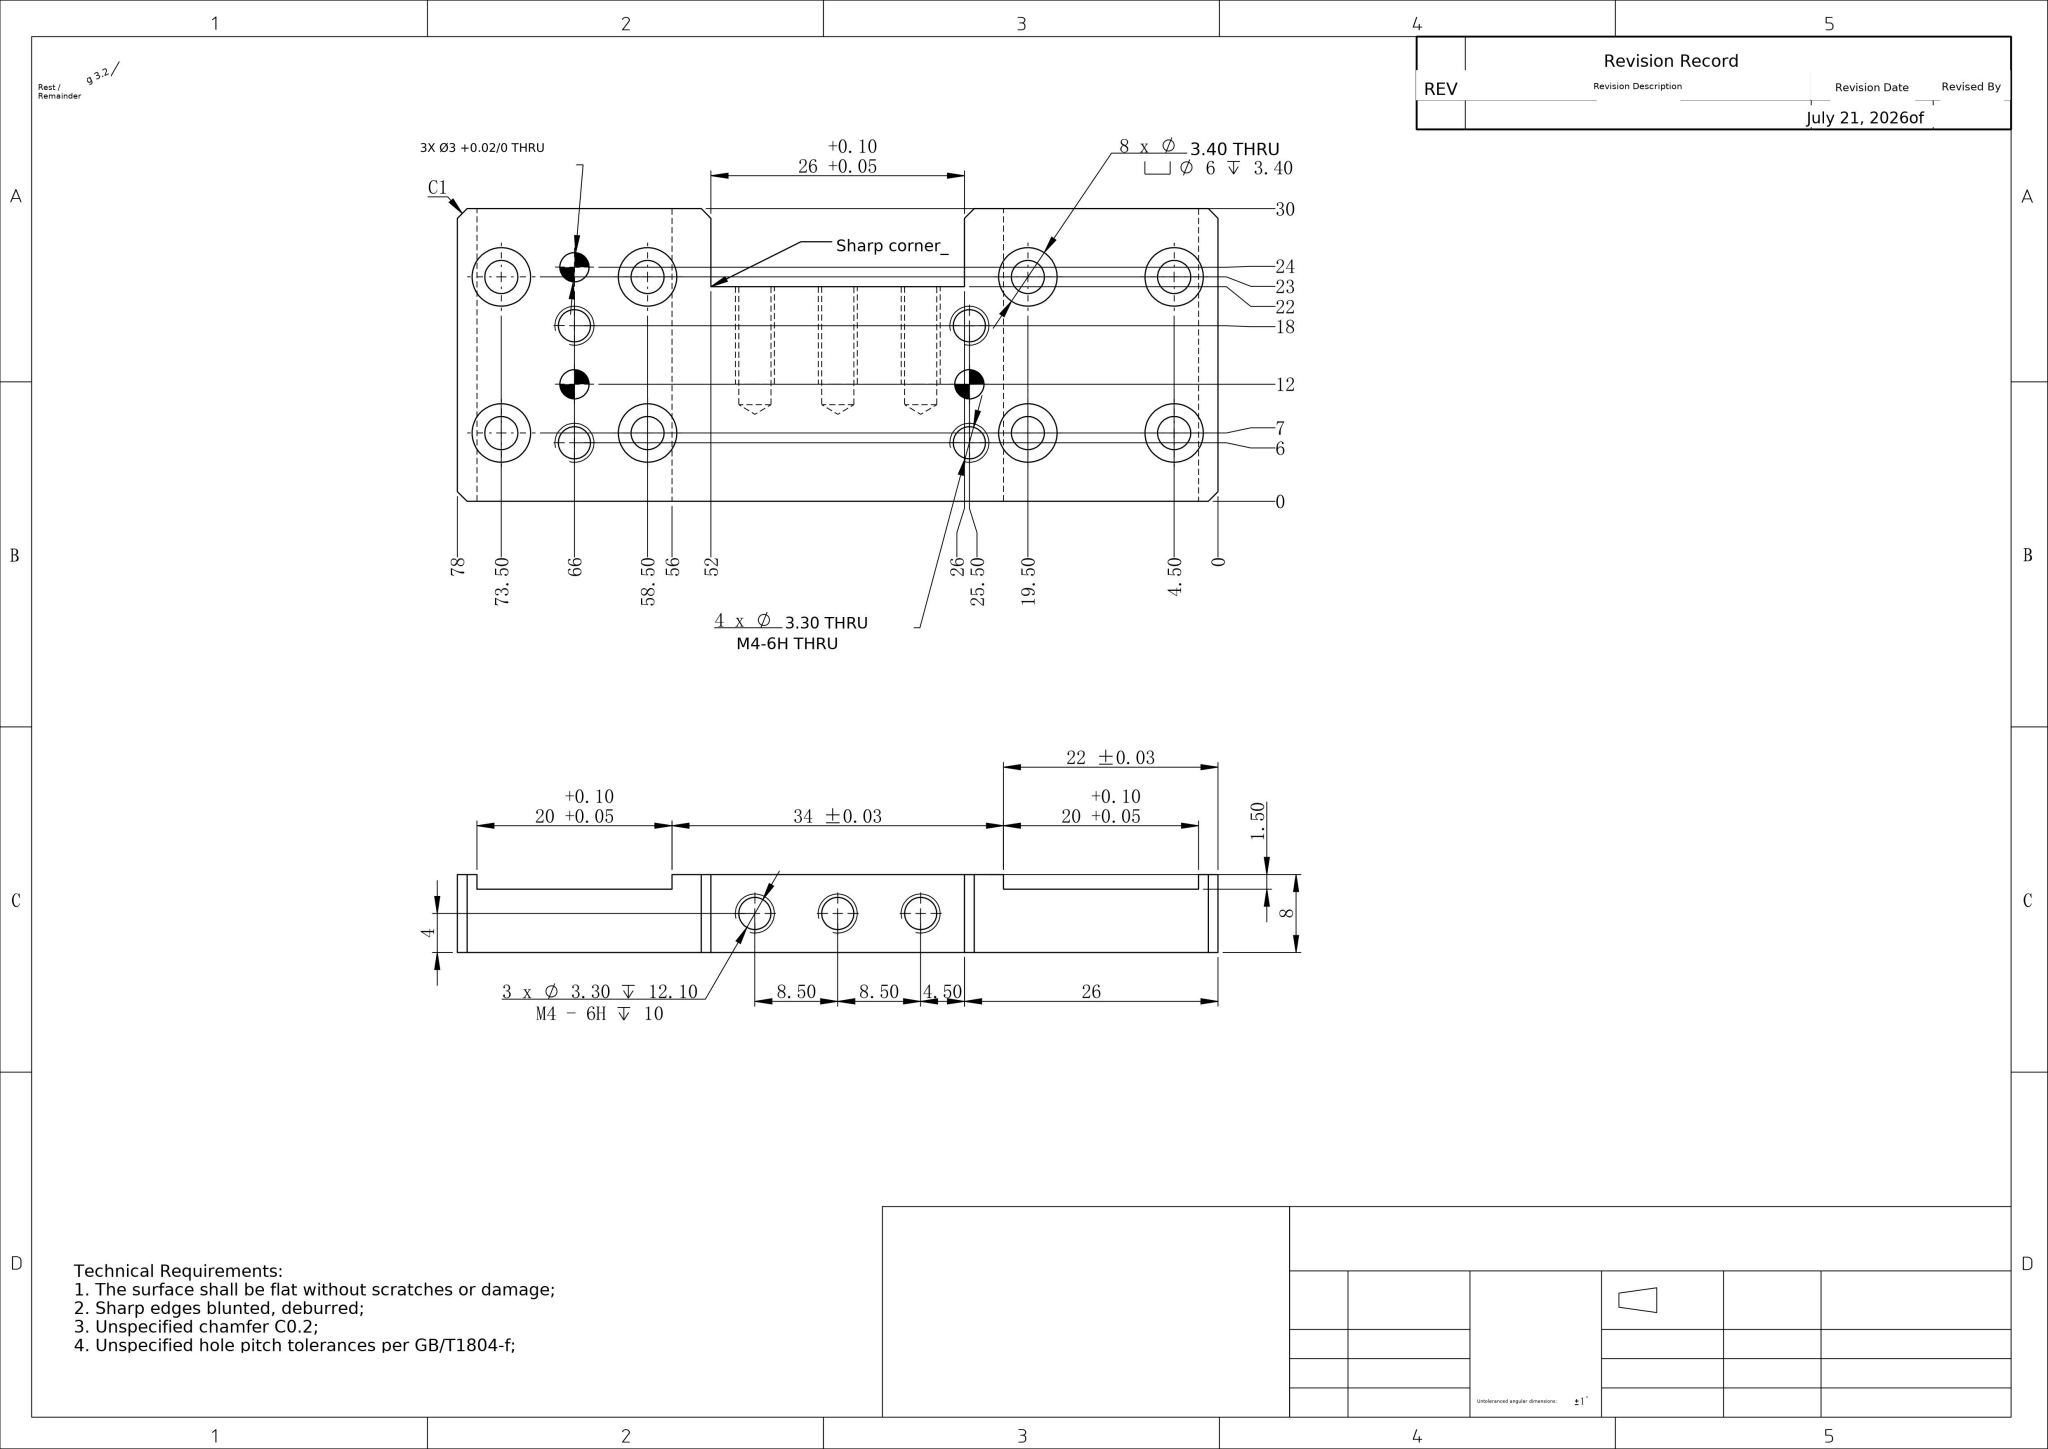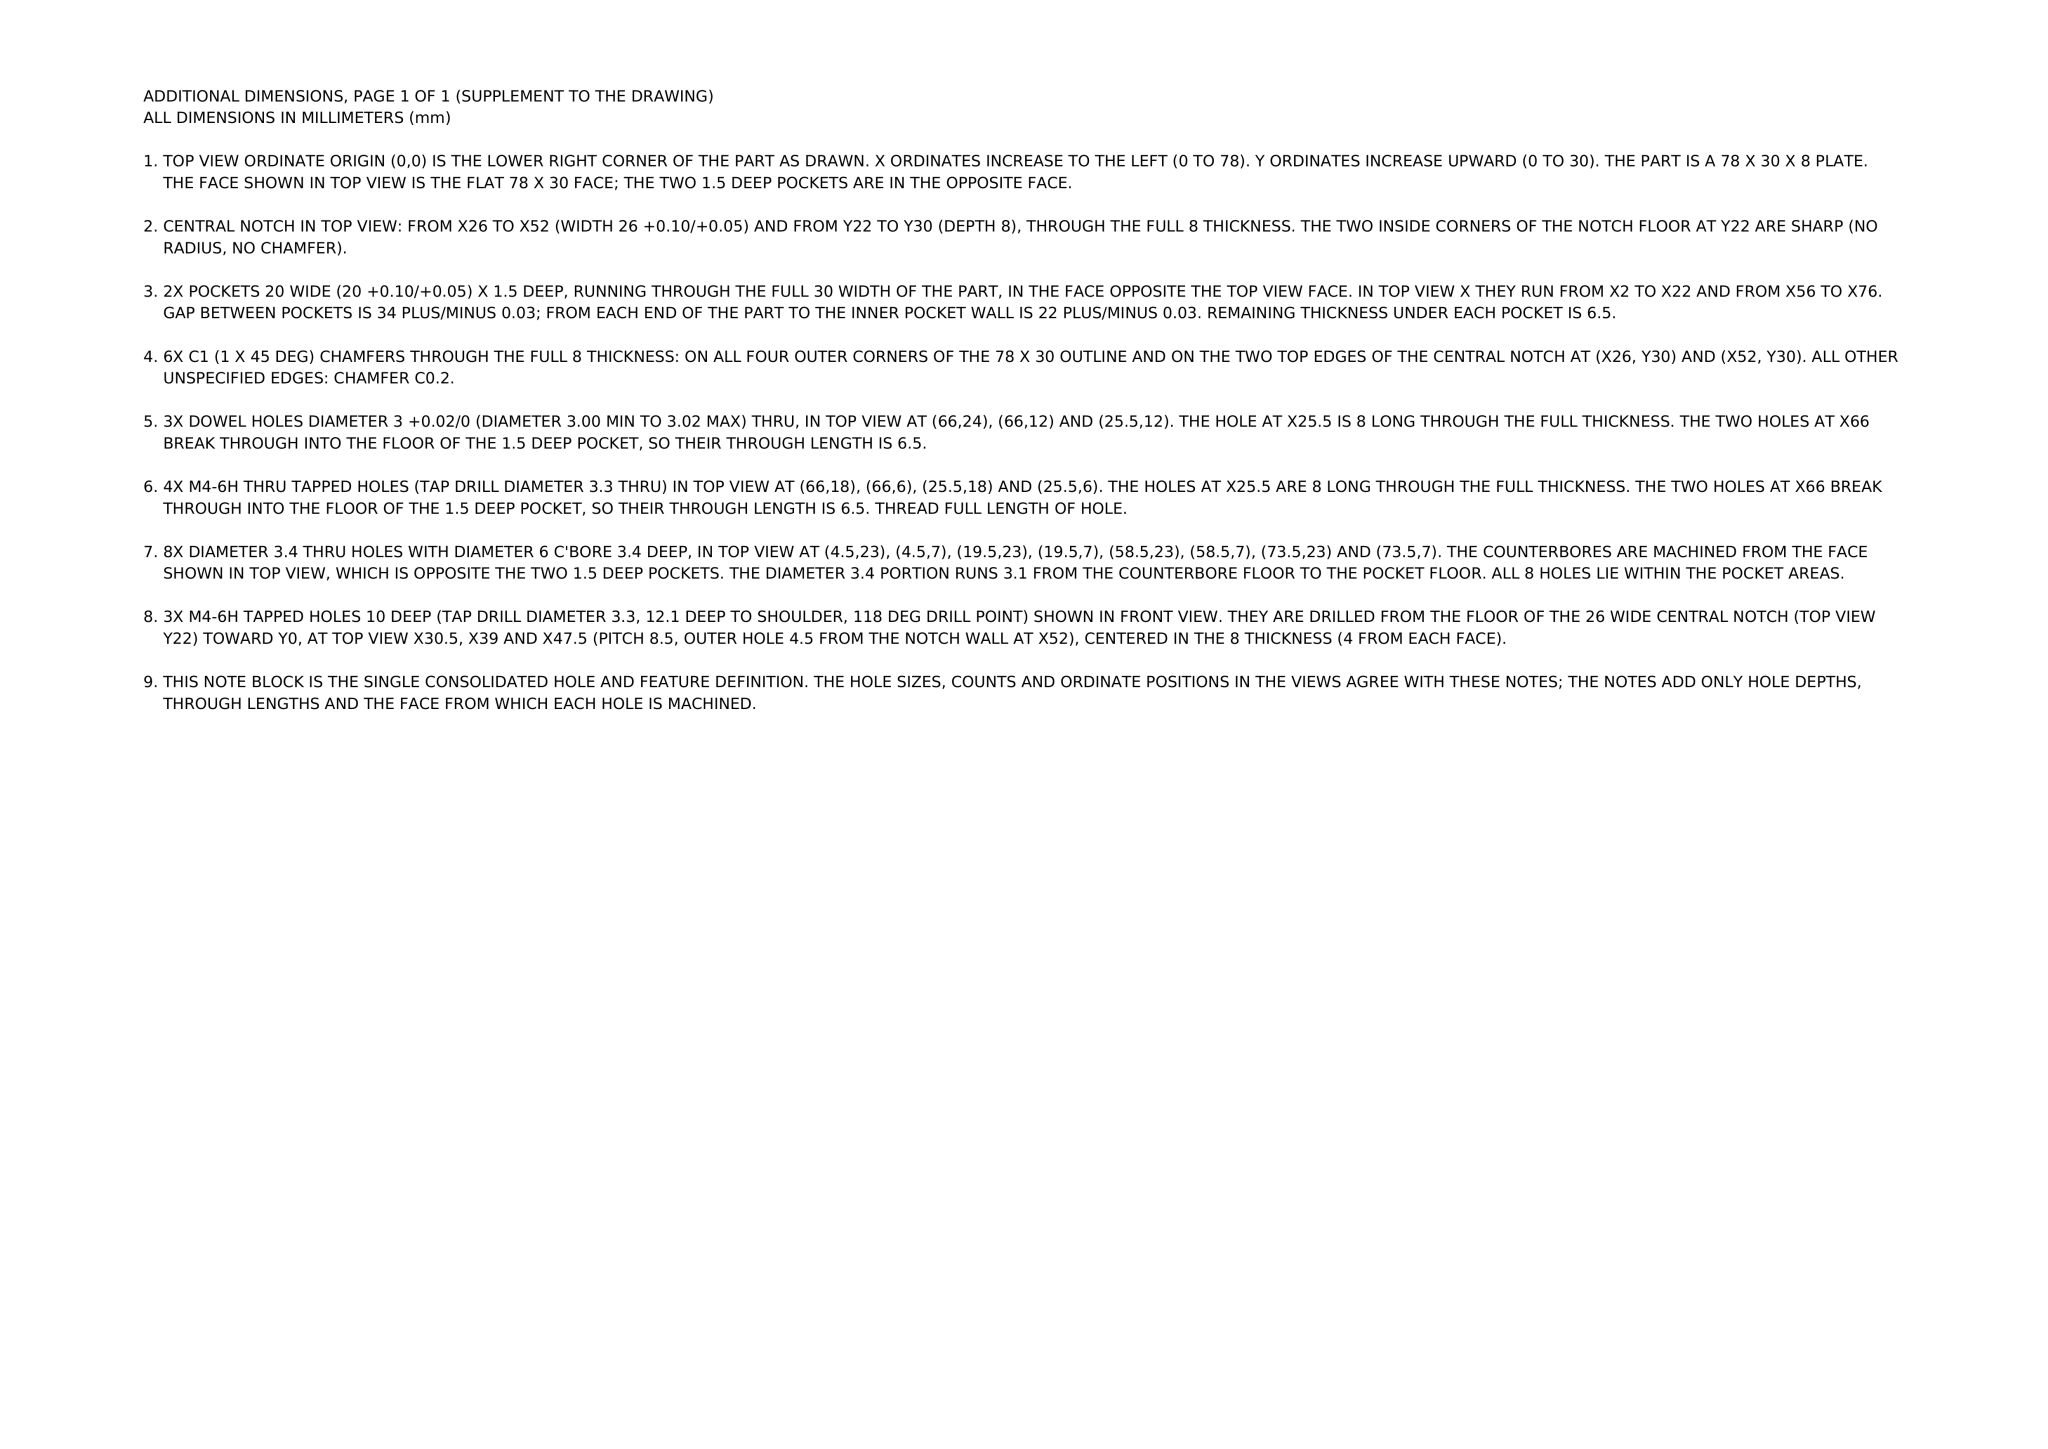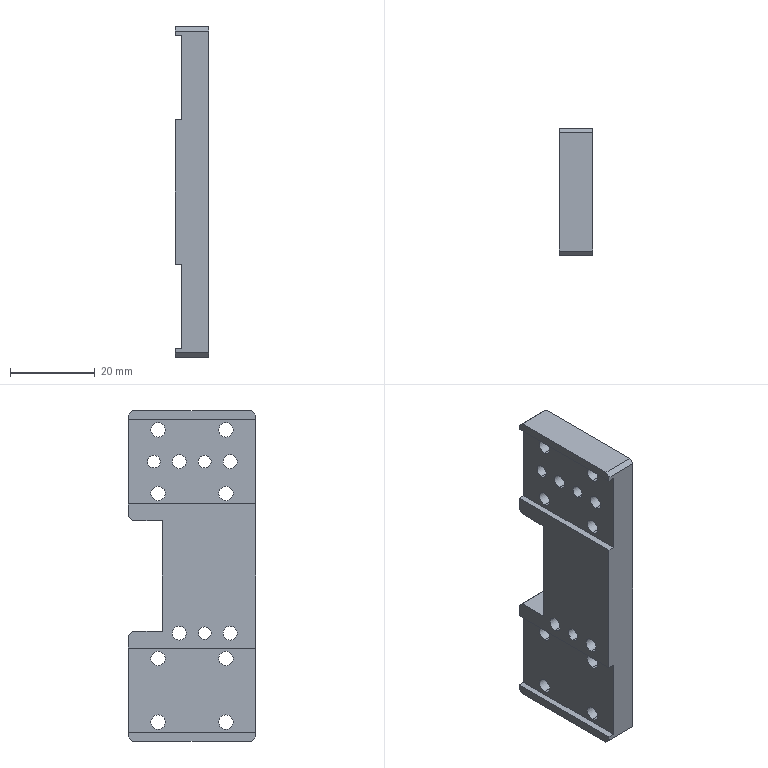Part | NX | mm | 1 solid | 90 faces | box 8 x 30 x 78 mm | volume 13522 mm3 | cylinder 52 | plane 32 | cone 6 | commonest cylinder face diameters 6 x16 3.4 x16 3.3 x14 3 x6